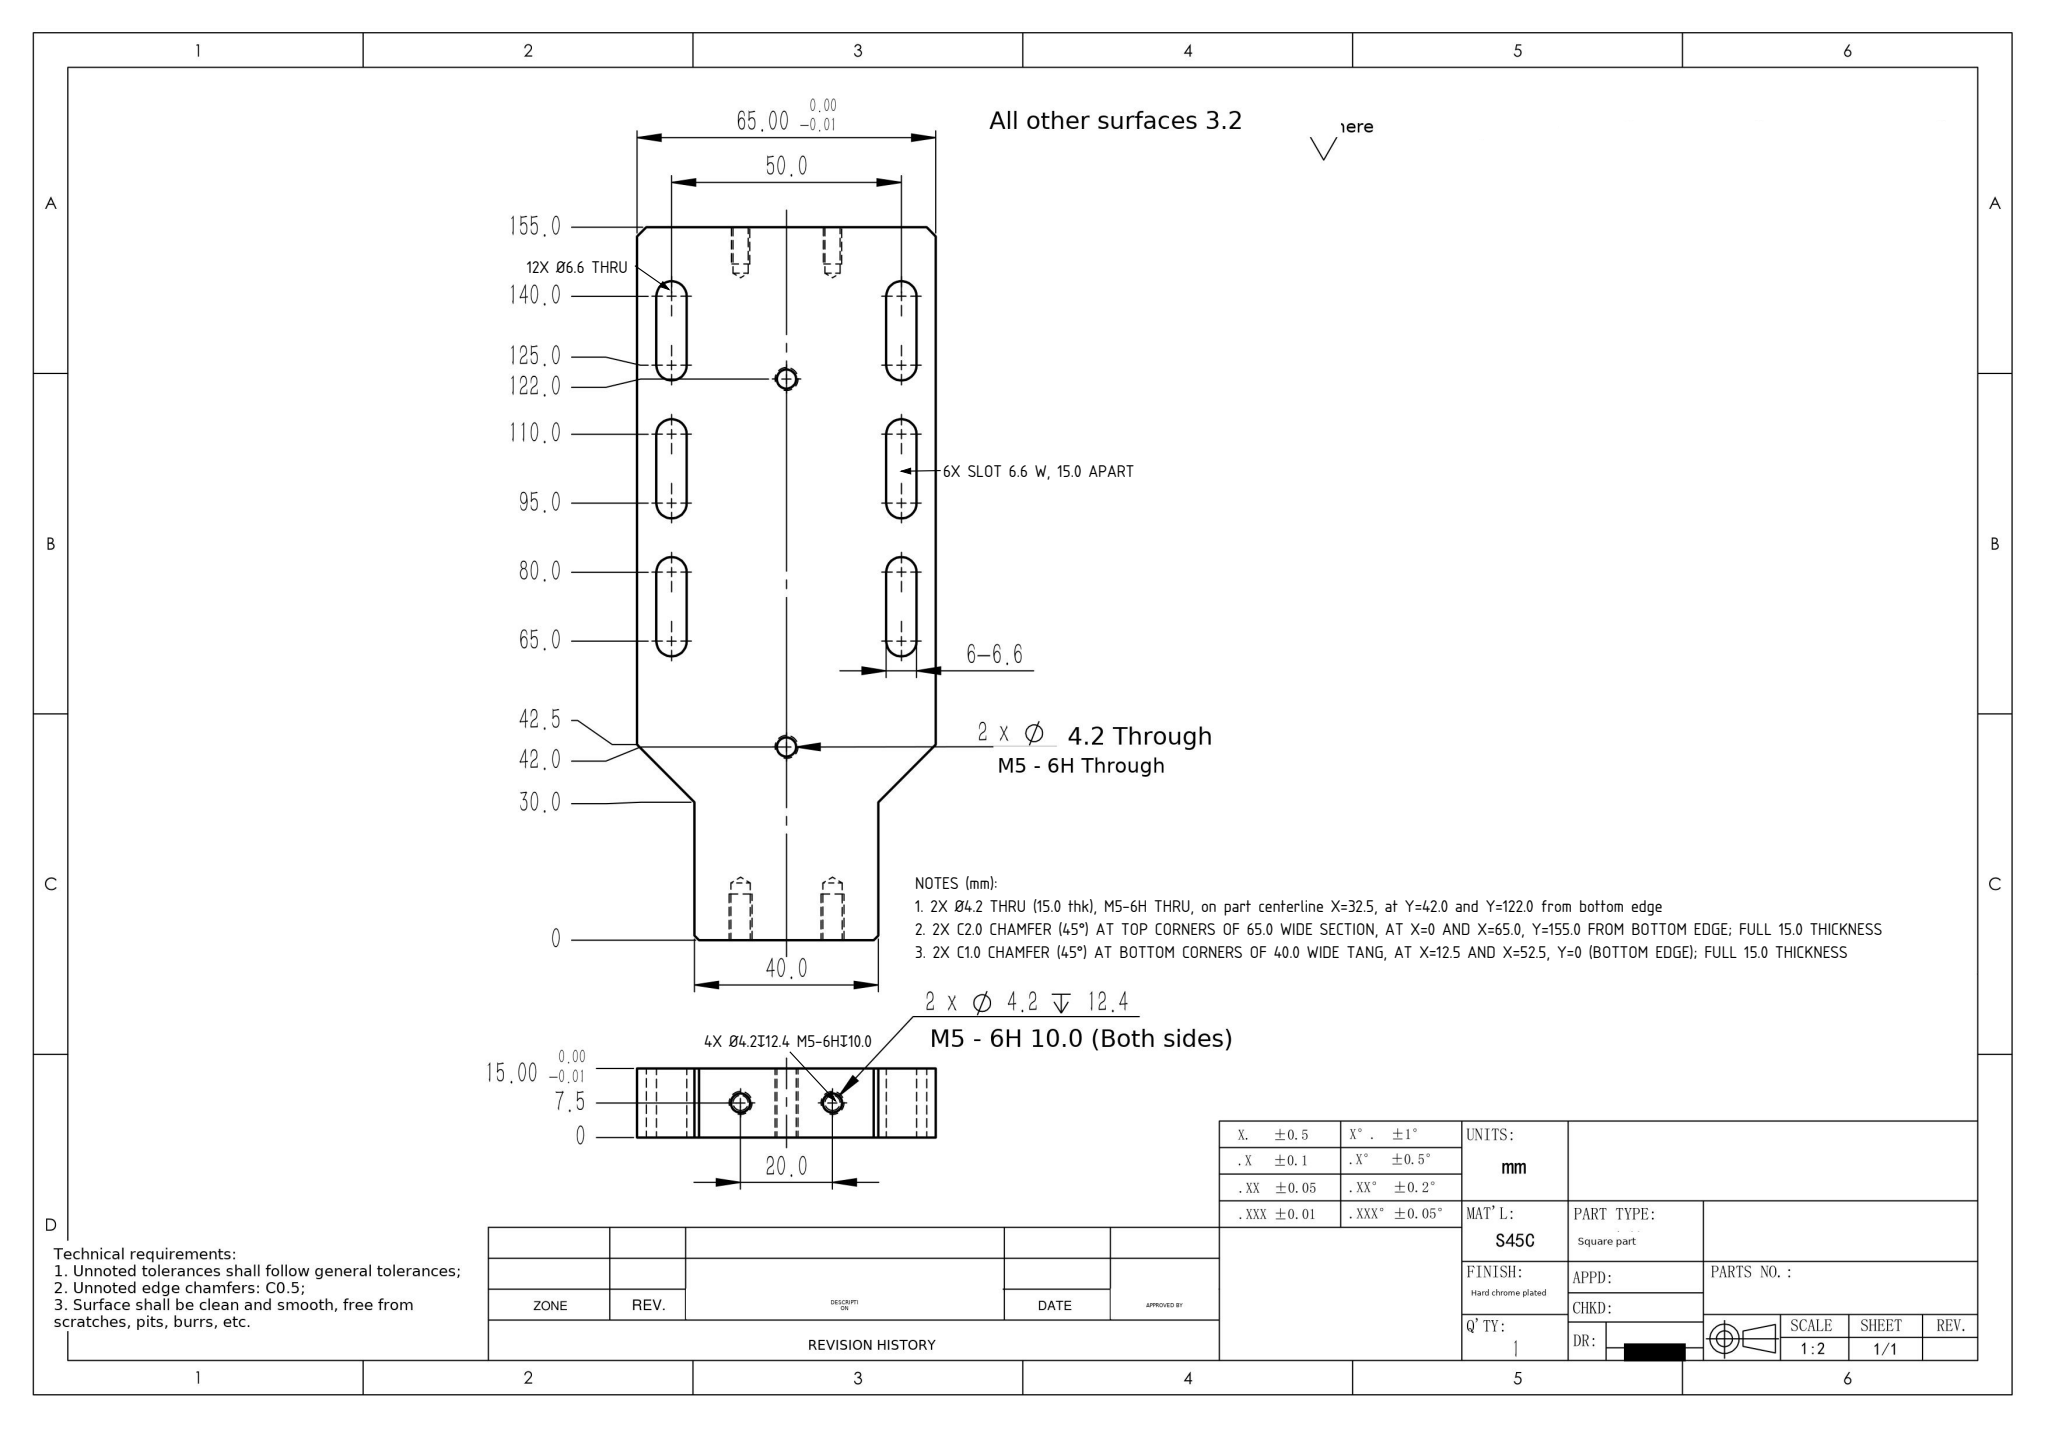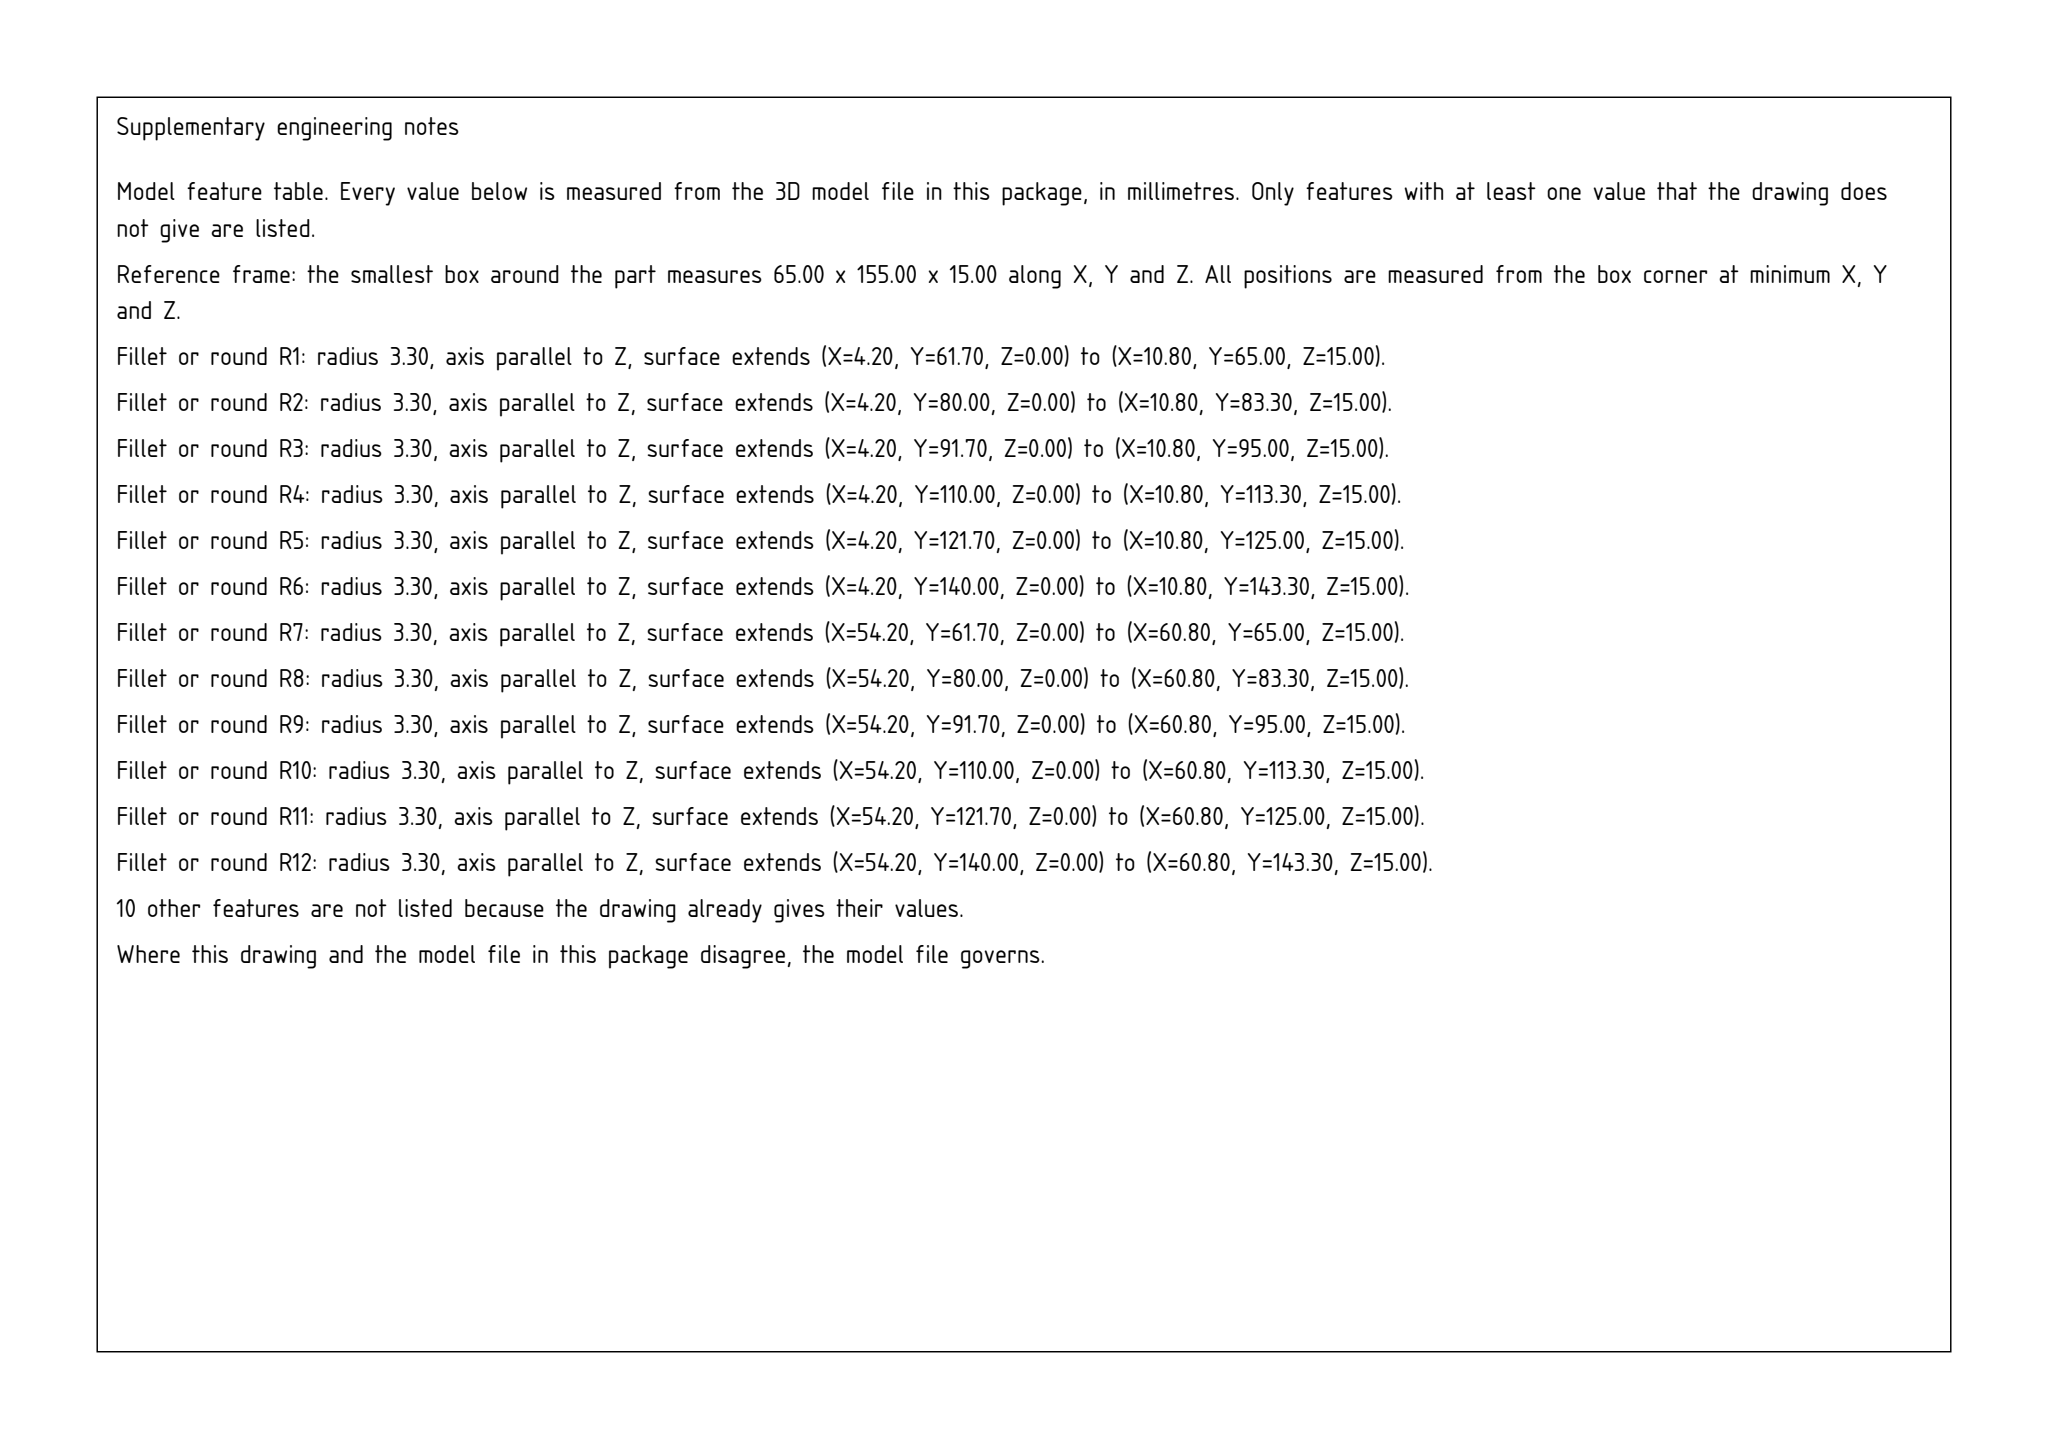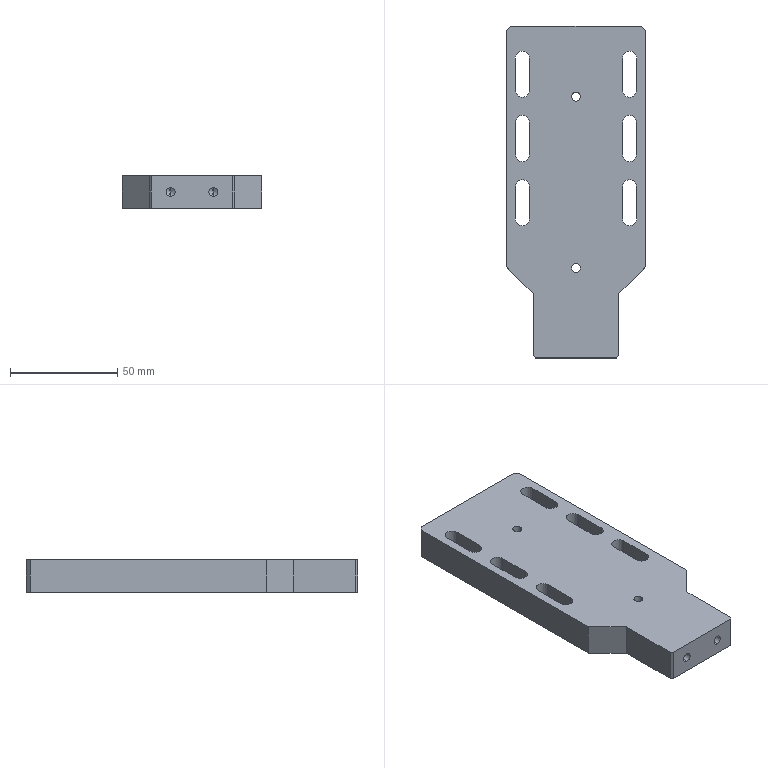Part | SolidWorks | mm | material S45C | 1 solid | 58 faces | box 65 x 155 x 15 mm | volume 124520 mm3 | plane 26 | cylinder 24 | cone 8 | commonest cylinder face diameters 6.6 x12 4.2 x8 3.3 x4
Drawing notes:
12X Ø6.6 THRU (15.0 thk), forming 6 slots; hole centers at X=7.5 and X=57.5 from left edge, Y=65.0, 80.0, 95.0, 110.0, 125.0, 140.0 from bottom edge | from the solid: cylinders dia 6.6, axis z, pos (7.5 & 57.5, 65/80/95/110/125/140), length 15.0, 12 total
2X Ø4.2 THRU (15.0 thk), M5-6H THRU, on part centerline X=32.5, at Y=42.0 and Y=122.0 from bottom edge | from the solid: cylinders dia 4.2, axis z, pos (32.5, 42.0) and (32.5, 122.0), length 15.0
4X Ø4.2 DP 12.4, M5-6H DP 10.0, in both 65.0 x 15.0 end faces (Y=0 and Y=155.0); holes at X=22.5 and X=42.5, Z=7.5 | from the solid: cylinders dia 4.2 and 3.3, axis y, pos (22.5 & 42.5, -, 7.5), lengths 12.4 and 10.0, 2 each
6X SLOT 6.6 WIDE (formed by Ø6.6 THRU end holes 15.0 APART), 3 PER SIDE; HOLE CENTERS AT X=7.5 AND X=57.5 FROM LEFT EDGE, Y=65.0/80.0, 95.0/110.0, 125.0/140.0 FROM BOTTOM EDGE | from the solid: cylinders dia 6.6, axis z, length 15.0 at (7.5 and 57.5, y=65/80/95/110/125/140)
2X C2.0 CHAMFER (45°) AT TOP CORNERS OF 65.0 WIDE SECTION, AT X=0 AND X=65.0, Y=155.0 FROM BOTTOM EDGE; FULL 15.0 THICKNESS | from the solid: inclined_planes: 45°/45°/90° at bbox_from [0.0,153.0,0.0] and [63.0,153.0,0.0], size [2.0,2.0,15.0]
2X C1.0 CHAMFER (45°) AT BOTTOM CORNERS OF 40.0 WIDE TANG, AT X=12.5 AND X=52.5, Y=0 (BOTTOM EDGE); FULL 15.0 THICKNESS | from the solid: inclined_planes: 45°/45°/90° at bbox_from [12.5,0.0,0.0] and [51.5,0.0,0.0], size [1.0,1.0,15.0]